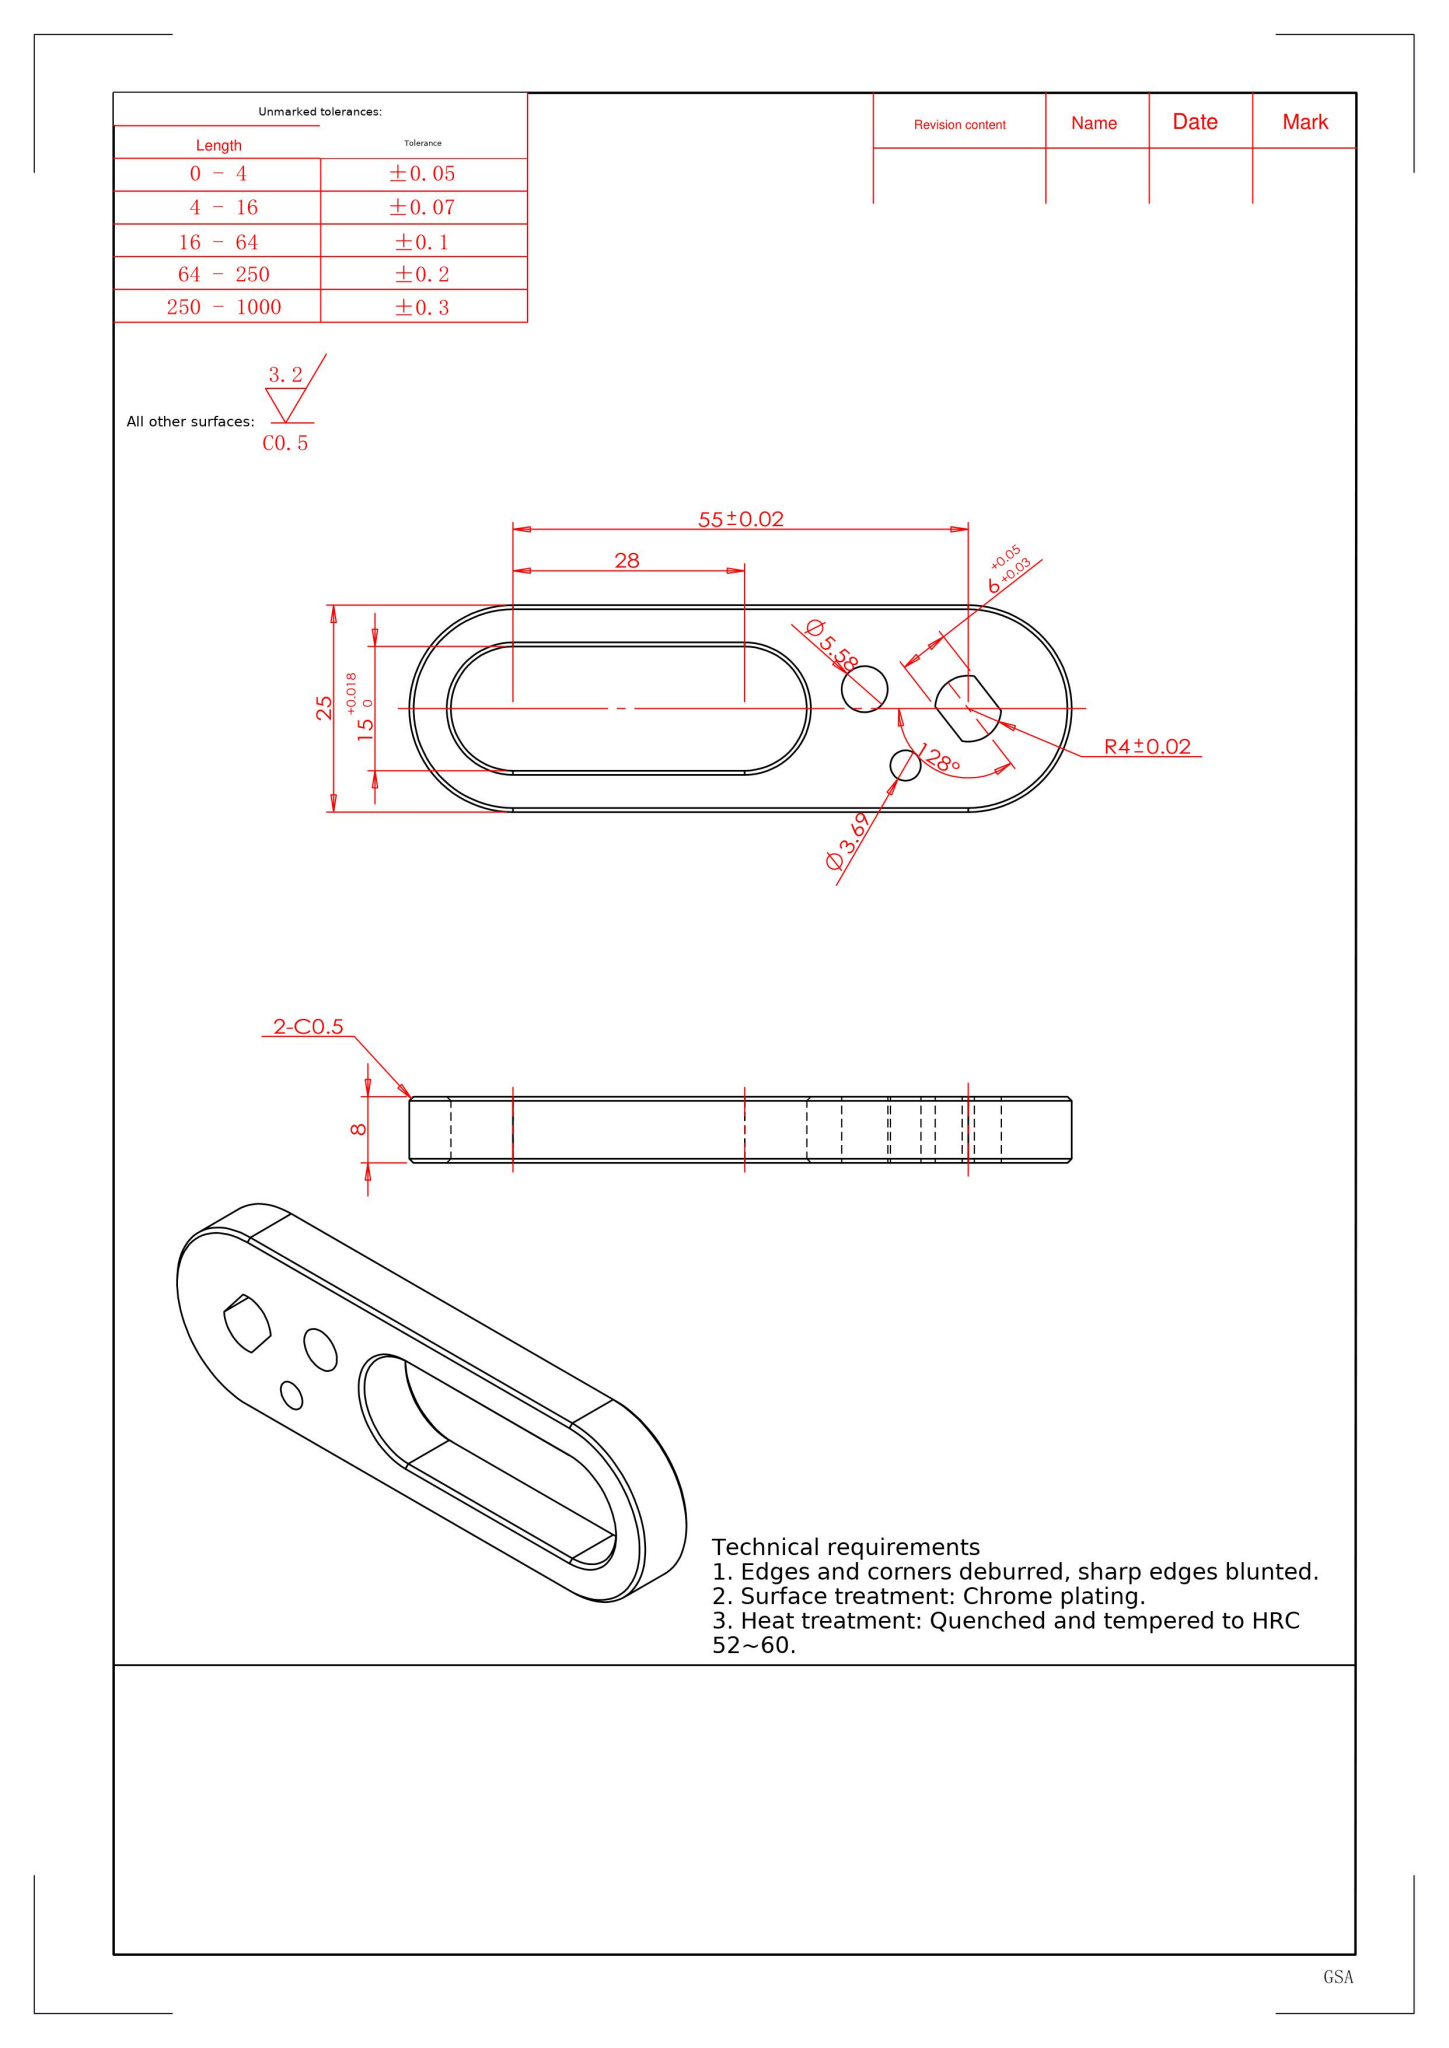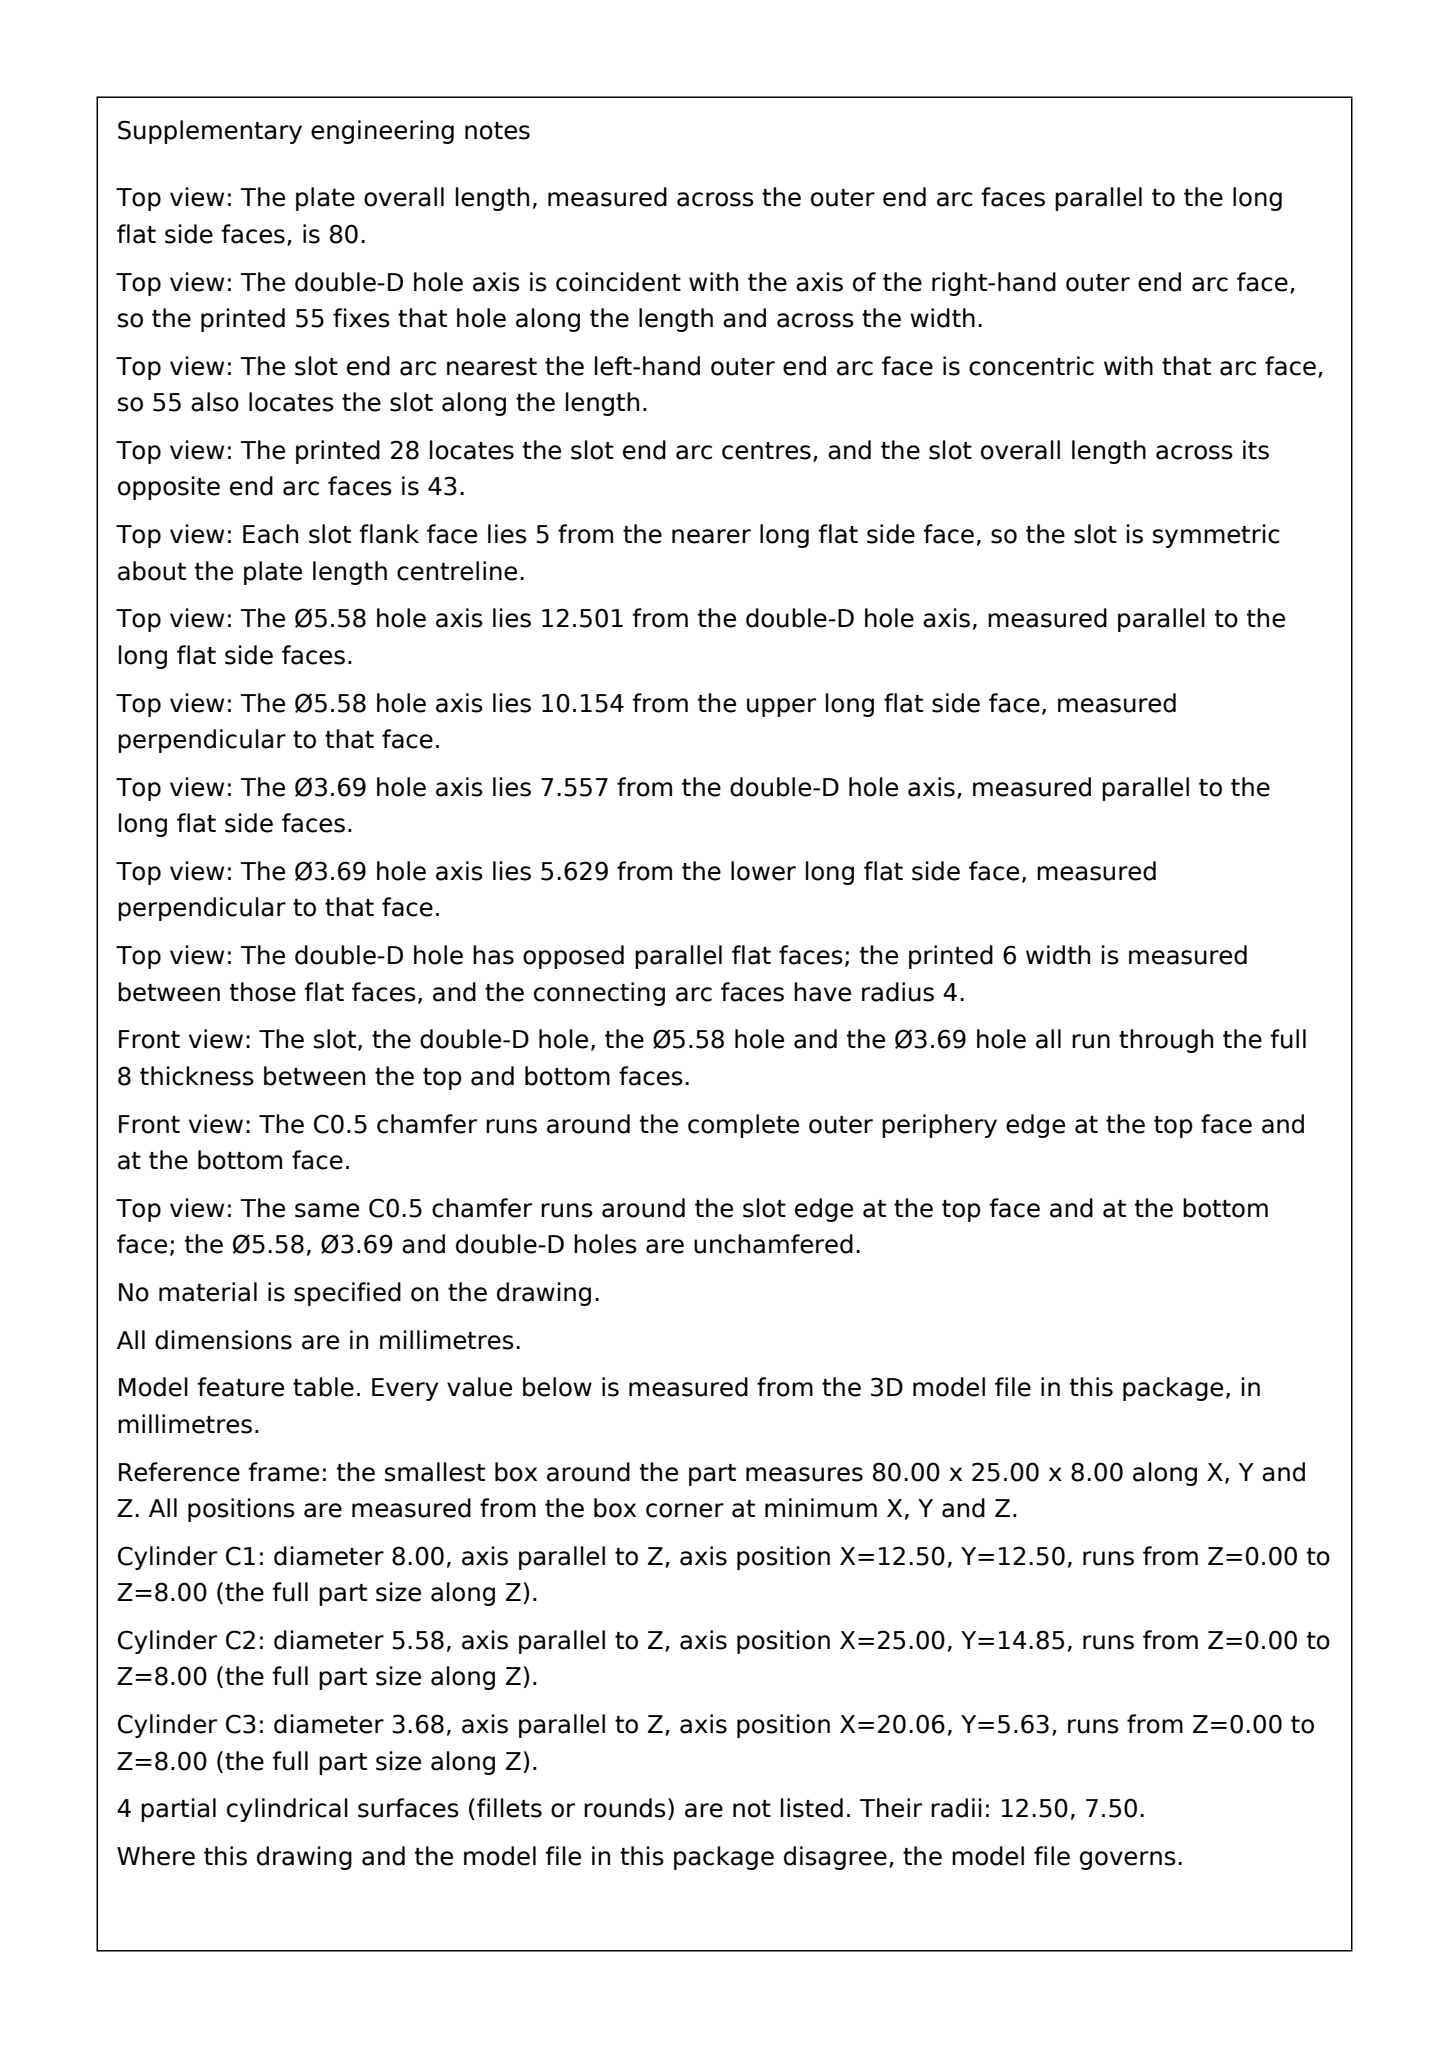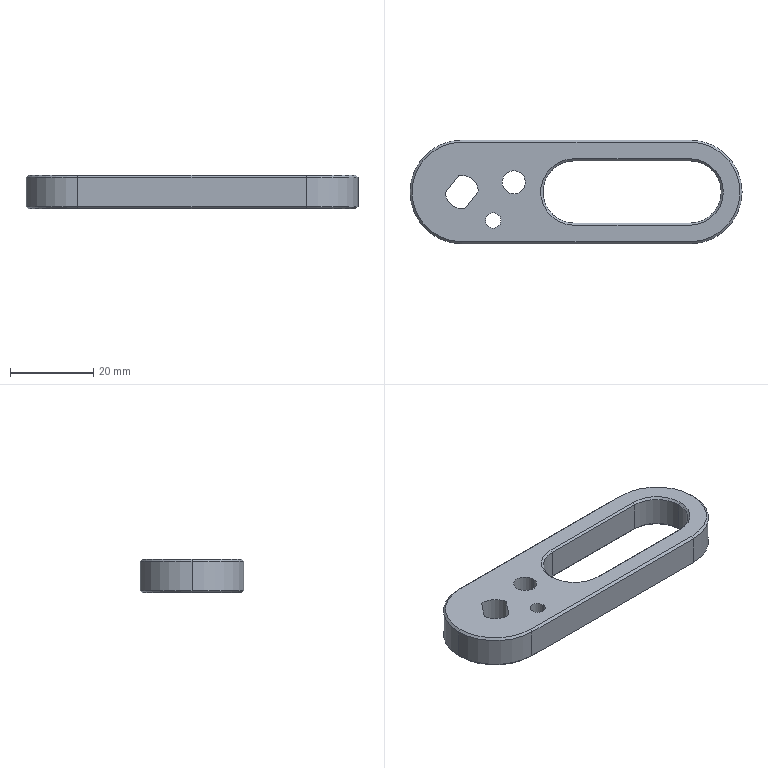Part | SolidWorks | mm | 1 solid | 40 faces | box 80 x 25 x 8 mm | volume 9455 mm3 | plane 16 | cylinder 12 | cone 12 | commonest cylinder face diameters 15 x3 25 x3 5.578 x2 3.687 x2 8 x2
Drawing notes:
POLYGON HOLE THRU 8 THK: ENVELOPE Ø8, AXIS AT X=12.5 FROM LEFT END FACE, Y=12.5 FROM LONG EDGE (ON PART CL) | from the solid: cylinders: concave arc dia 8.0, axis z at [12.5,12.5], from 0.0 to 8.0 (full 8 thk)
POLYGON HOLE CLOCKING: TWO FLAT FACES, EACH FULL 8 THK, INCLINED 38° TO X AXIS (PART CL) AND 52° TO Y AXIS; FLATS AT X=8.5-11.8 / Y=12.3-16.5 AND X=13.2-16.5 / Y=8.6-12.8 FROM MIN CORNER | from the solid: inclined_planes: angle_to_xyz_axes [38,52,90], bbox_from [8.5,12.3,0] size [3.3,4.2,8] and bbox_from [13.2,8.6,0] size [3.3,4.2,8]
REMAINDER OF POLYGON HOLE WALL IS A SINGLE Ø8 ARC FACE OF 194° SWEEP, CENTERED ON THE HOLE AXIS AT X=12.5, Y=12.5 | from the solid: cylinders: concave arc dia 8.0, axis z [12.5,12.5], arc_deg 194
SLOT 15 WIDE x 28 LG, R7.5 ENDS, THRU FULL 8 THK (NO FLOOR); END ARC CTRS ON PART CL Y=12.5, AT X=39.5 AND X=67.5 FROM LEFT END FACE | from the solid: concave arc dia 15, axis z at (39.5,12.5) and (67.5,12.5), from z=0.5 to 7.5, 180 deg; planes normal y at y=5.0 and y=20.0, extent x 39.5-67.5, z 0.5-7.5; no z-normal floor face inside slot (only z=0 and z=8 outer faces)
SLOT EDGES: C0.5 CHAMFER ON BOTH FACES (z=0 AND z=8) ALL ROUND, 28 LG ALONG EACH SLOT SIDE | from the solid: inclined planes 45 deg, bbox_from [39.5,20.0,0.0], [39.5,20.0,7.5], [39.5,4.5,0.0], [39.5,4.5,7.5], size [28.0,0.5,0.5]
build123d program:
from build123d import *

# Parameters (mm, degrees)
BOSS_EXTRUDE1_DEPTH = 8
CUT_EXTRUDE1_DEPTH  = 43.664
SKETCH3_R           = 4
CUT_EXTRUDE2_DEPTH  = 43.664
BOSS_EXTRUDE2_START = -8
BOSS_EXTRUDE2_DEPTH = 8
CHAMFER1_SIZE       = 0.5
SKETCH5_R           = 2.789
SKETCH5_R_2         = 1.843
CUT_EXTRUDE3_DEPTH  = 10


with BuildPart() as part:
    # Sketch1 → Boss-Extrude1 (new body)
    with BuildSketch(Plane.XY):
        with BuildLine():
            Line((-27.5, 12.5), (27.5, 12.5))
            ThreePointArc((27.5, 12.5), (40, 0), (27.5, -12.5))
            Line((27.5, -12.5), (-27.5, -12.5))
            ThreePointArc((-27.5, -12.5), (-40, 0), (-27.5, 12.5))
        make_face()
    extrude(amount=BOSS_EXTRUDE1_DEPTH)

    # Sketch2 → Cut-Extrude1 (cut, through all)
    with BuildSketch(Plane.XY.offset(8)):
        with BuildLine():
            Line((-0.5, 7.5), (27.5, 7.5))
            ThreePointArc((27.5, 7.5), (35, 0), (27.5, -7.5))
            Line((27.5, -7.5), (-0.5, -7.5))
            ThreePointArc((-0.5, -7.5), (-8, 0), (-0.5, 7.5))
        make_face()
    extrude(amount=-CUT_EXTRUDE1_DEPTH, mode=Mode.SUBTRACT)

    # Sketch3 → Cut-Extrude2 (cut, through all)
    with BuildSketch(Plane.XY.offset(8)):
        with Locations((-27.5, 0)):
            Circle(SKETCH3_R)
    extrude(amount=-CUT_EXTRUDE2_DEPTH, mode=Mode.SUBTRACT)

    # Sketch4 → Boss-Extrude2 (add)
    with BuildSketch(Plane(origin=(0, 0, 0), x_dir=(-1, 0, 0), z_dir=(0, 0, -1)).offset(BOSS_EXTRUDE2_START)):
        with BuildLine():
            Line((23.507, 0.2379), (26.765, -3.932))
            ThreePointArc((26.765, -3.932), (24.348, -2.463), (23.507, 0.2379))
        make_face()
        with BuildLine():
            Line((28.235, 3.932), (31.493, -0.2379))
            ThreePointArc((31.493, -0.2379), (30.652, 2.463), (28.235, 3.932))
        make_face()
    extrude(amount=BOSS_EXTRUDE2_DEPTH)

    # Chamfer1
    chamfer1_edges = [part.edges().sort_by_distance(p)[0] for p in [
        (40, 0, 8),
        (0, 12.5, 8),
        (-8, 0, 0),
        (13.5, 7.5, 0),
        (35, 0, 0),
        (13.5, -7.5, 0),
        (-8, 0, 8),
        (13.5, -7.5, 8),
        (35, 0, 8),
        (13.5, 7.5, 8),
        (-40, 0, 8),
        (0, 12.5, 0),
        (40, 0, 0),
        (0, -12.5, 0),
        (-40, 0, 0),
        (0, -12.5, 8),
    ]]
    chamfer(chamfer1_edges, length=CHAMFER1_SIZE)

    # Sketch5 → Cut-Extrude3 (cut)
    with BuildSketch(Plane(origin=(0, 0, 0), x_dir=(-1, 0, 0), z_dir=(0, 0, -1))):
        with Locations((14.999, 2.346)):
            Circle(SKETCH5_R)
        with Locations((19.943, -6.871)):
            Circle(SKETCH5_R_2)
    extrude(amount=-CUT_EXTRUDE3_DEPTH, mode=Mode.SUBTRACT)


solid = part.part